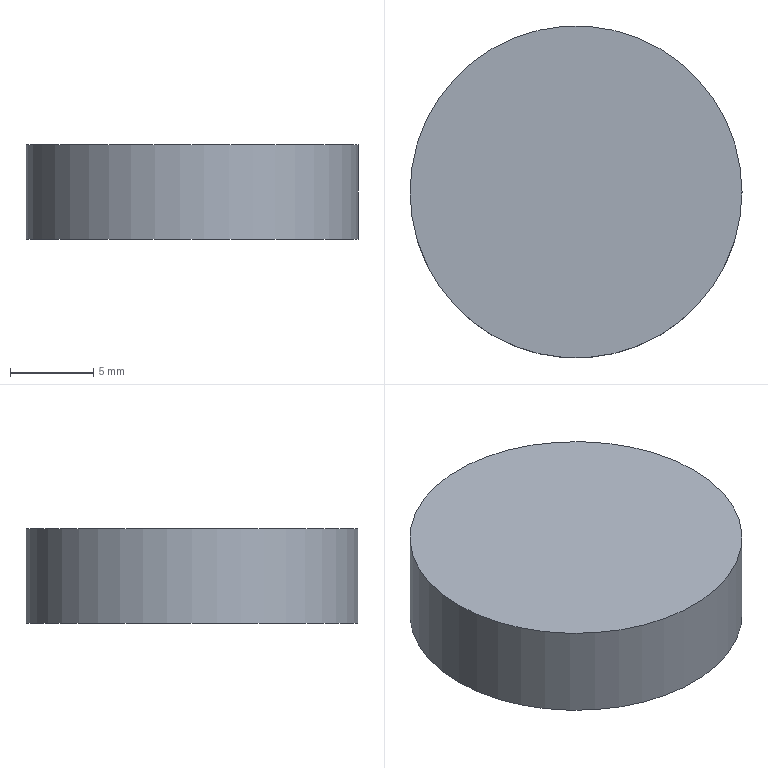Component | NX | ATOMIZER_HEAD | 1 solid | 3 faces | box 20 x 20 x 5.68 mm | volume 1784 mm3 | plane 2 | cylinder 1 | commonest cylinder face diameters 20 x1
STEP:
#1=CARTESIAN_POINT('',(0.,0.,0.));
#2=DIRECTION('',(0.,0.,1.));
#3=DIRECTION('',(1.,0.,0.));
#4=AXIS2_PLACEMENT_3D('',#1,#2,#3);
#5=CARTESIAN_POINT('',(-11.276,33.197,23.456));
#6=VERTEX_POINT('',#5);
#7=CARTESIAN_POINT('',(-21.276,33.197,23.456));
#8=DIRECTION('',(0.,0.,-1.));
#9=DIRECTION('',(1.,0.,0.));
#10=AXIS2_PLACEMENT_3D('',#7,#8,#9);
#11=CIRCLE('',#10,10.);
#12=CARTESIAN_POINT('',(-21.276,33.197,23.456));
#13=DIRECTION('',(0.,0.,1.));
#14=DIRECTION('',(1.,0.,0.));
#15=AXIS2_PLACEMENT_3D('',#12,#13,#14);
#16=PLANE('',#15);
#17=CARTESIAN_POINT('',(10.,0.));
#18=CARTESIAN_POINT('',(10.,-17.321));
#19=CARTESIAN_POINT('',(-5.,-8.66));
#20=CARTESIAN_POINT('',(-20.,-0.));
#21=CARTESIAN_POINT('',(-5.,8.66));
#22=CARTESIAN_POINT('',(10.,17.321));
#23=CARTESIAN_POINT('',(10.,0.));
#24=(BOUNDED_CURVE()B_SPLINE_CURVE(2,(#17,#18,#19,#20,#21,#22,#23),.UNSPECIFIED.,.T.,.F.)B_SPLINE_CURVE_WITH_KNOTS((1,2,2,2,2,1),(-2.094,0.,2.094,4.189,6.283,8.378),.UNSPECIFIED.)CURVE()GEOMETRIC_REPRESENTATION_ITEM()RATIONAL_B_SPLINE_CURVE((1.,0.5,1.,0.5,1.,0.5,1.))REPRESENTATION_ITEM(''));
#25=(GEOMETRIC_REPRESENTATION_CONTEXT(2)PARAMETRIC_REPRESENTATION_CONTEXT()REPRESENTATION_CONTEXT('',''));
#26=DEFINITIONAL_REPRESENTATION('',(#24),#25);
#27=PCURVE('',#16,#26);
#28=CARTESIAN_POINT('',(-21.276,33.197,17.776));
#29=DIRECTION('',(0.,0.,1.));
#30=DIRECTION('',(1.,0.,0.));
#31=AXIS2_PLACEMENT_3D('',#28,#29,#30);
#32=CYLINDRICAL_SURFACE('',#31,10.);
#33=CARTESIAN_POINT('',(6.283,5.68));
#34=DIRECTION('',(-1.,0.));
#35=VECTOR('',#34,1.);
#36=LINE('',#33,#35);
#37=(GEOMETRIC_REPRESENTATION_CONTEXT(2)PARAMETRIC_REPRESENTATION_CONTEXT()REPRESENTATION_CONTEXT('',''));
#38=DEFINITIONAL_REPRESENTATION('',(#36),#37);
#39=PCURVE('',#32,#38);
#40=SURFACE_CURVE('',#11,(#27,#39),.PCURVE_S1.);
#41=EDGE_CURVE('',#6,#6,#40,.T.);
#42=ORIENTED_EDGE('',*,*,#41,.F.);
#43=EDGE_LOOP('',(#42));
#44=FACE_BOUND('',#43,.T.);
#45=ADVANCED_FACE('',(#44),#16,.T.);
#46=CARTESIAN_POINT('',(-11.276,33.197,17.776));
#47=VERTEX_POINT('',#46);
#48=CARTESIAN_POINT('',(-21.276,33.197,17.776));
#49=DIRECTION('',(0.,0.,1.));
#50=DIRECTION('',(1.,0.,0.));
#51=AXIS2_PLACEMENT_3D('',#48,#49,#50);
#52=CIRCLE('',#51,10.);
#53=CARTESIAN_POINT('',(-21.276,33.197,17.776));
#54=DIRECTION('',(0.,0.,-1.));
#55=DIRECTION('',(-1.,0.,0.));
#56=AXIS2_PLACEMENT_3D('',#53,#54,#55);
#57=PLANE('',#56);
#58=CARTESIAN_POINT('',(-10.,0.));
#59=CARTESIAN_POINT('',(-10.,17.321));
#60=CARTESIAN_POINT('',(5.,8.66));
#61=CARTESIAN_POINT('',(20.,0.));
#62=CARTESIAN_POINT('',(5.,-8.66));
#63=CARTESIAN_POINT('',(-10.,-17.321));
#64=CARTESIAN_POINT('',(-10.,0.));
#65=(BOUNDED_CURVE()B_SPLINE_CURVE(2,(#58,#59,#60,#61,#62,#63,#64),.UNSPECIFIED.,.T.,.F.)B_SPLINE_CURVE_WITH_KNOTS((1,2,2,2,2,1),(-2.094,0.,2.094,4.189,6.283,8.378),.UNSPECIFIED.)CURVE()GEOMETRIC_REPRESENTATION_ITEM()RATIONAL_B_SPLINE_CURVE((1.,0.5,1.,0.5,1.,0.5,1.))REPRESENTATION_ITEM(''));
#66=(GEOMETRIC_REPRESENTATION_CONTEXT(2)PARAMETRIC_REPRESENTATION_CONTEXT()REPRESENTATION_CONTEXT('',''));
#67=DEFINITIONAL_REPRESENTATION('',(#65),#66);
#68=PCURVE('',#57,#67);
#69=CARTESIAN_POINT('',(0.,0.));
#70=DIRECTION('',(1.,0.));
#71=VECTOR('',#70,1.);
#72=LINE('',#69,#71);
#73=(GEOMETRIC_REPRESENTATION_CONTEXT(2)PARAMETRIC_REPRESENTATION_CONTEXT()REPRESENTATION_CONTEXT('',''));
#74=DEFINITIONAL_REPRESENTATION('',(#72),#73);
#75=PCURVE('',#32,#74);
#76=SURFACE_CURVE('',#52,(#68,#75),.PCURVE_S1.);
#77=EDGE_CURVE('',#47,#47,#76,.T.);
#78=ORIENTED_EDGE('',*,*,#77,.F.);
#79=EDGE_LOOP('',(#78));
#80=FACE_BOUND('',#79,.T.);
#81=ADVANCED_FACE('',(#80),#57,.T.);
#82=ORIENTED_EDGE('',*,*,#41,.T.);
#83=CARTESIAN_POINT('',(-11.276,33.197,17.776));
#84=CARTESIAN_POINT('',(-11.276,33.197,23.456));
#85=B_SPLINE_CURVE_WITH_KNOTS('',1,(#83,#84),.UNSPECIFIED.,.F.,.F.,(2,2),(0.,5.68),.PIECEWISE_BEZIER_KNOTS.);
#86=CARTESIAN_POINT('',(0.,0.));
#87=DIRECTION('',(0.,1.));
#88=VECTOR('',#87,1.);
#89=LINE('',#86,#88);
#90=(GEOMETRIC_REPRESENTATION_CONTEXT(2)PARAMETRIC_REPRESENTATION_CONTEXT()REPRESENTATION_CONTEXT('',''));
#91=DEFINITIONAL_REPRESENTATION('',(#89),#90);
#92=PCURVE('',#32,#91);
#93=CARTESIAN_POINT('',(6.283,0.));
#94=DIRECTION('',(0.,1.));
#95=VECTOR('',#94,1.);
#96=LINE('',#93,#95);
#97=(GEOMETRIC_REPRESENTATION_CONTEXT(2)PARAMETRIC_REPRESENTATION_CONTEXT()REPRESENTATION_CONTEXT('',''));
#98=DEFINITIONAL_REPRESENTATION('',(#96),#97);
#99=PCURVE('',#32,#98);
#100=SEAM_CURVE('',#85,(#92,#99),.PCURVE_S1.);
#101=EDGE_CURVE('',#47,#6,#100,.T.);
#102=ORIENTED_EDGE('',*,*,#101,.F.);
#103=ORIENTED_EDGE('',*,*,#77,.T.);
#104=ORIENTED_EDGE('',*,*,#101,.T.);
#105=EDGE_LOOP('',(#82,#102,#103,#104));
#106=FACE_BOUND('',#105,.T.);
#107=ADVANCED_FACE('',(#106),#32,.T.);
#108=CLOSED_SHELL('',(#45,#81,#107));
#109=MANIFOLD_SOLID_BREP('',#108);
#110=(LENGTH_UNIT()NAMED_UNIT(*)SI_UNIT(.MILLI.,.METRE.));
#111=UNCERTAINTY_MEASURE_WITH_UNIT(LENGTH_MEASURE(0.00001),#110,'','');
#112=(NAMED_UNIT(*)PLANE_ANGLE_UNIT()SI_UNIT($,.RADIAN.));
#113=(NAMED_UNIT(*)SI_UNIT($,.STERADIAN.)SOLID_ANGLE_UNIT());
#114=(GEOMETRIC_REPRESENTATION_CONTEXT(3)GLOBAL_UNCERTAINTY_ASSIGNED_CONTEXT((#111))GLOBAL_UNIT_ASSIGNED_CONTEXT((#110,#112,#113))REPRESENTATION_CONTEXT('',''));
#115=ADVANCED_BREP_SHAPE_REPRESENTATION('',(#4,#109),#114);